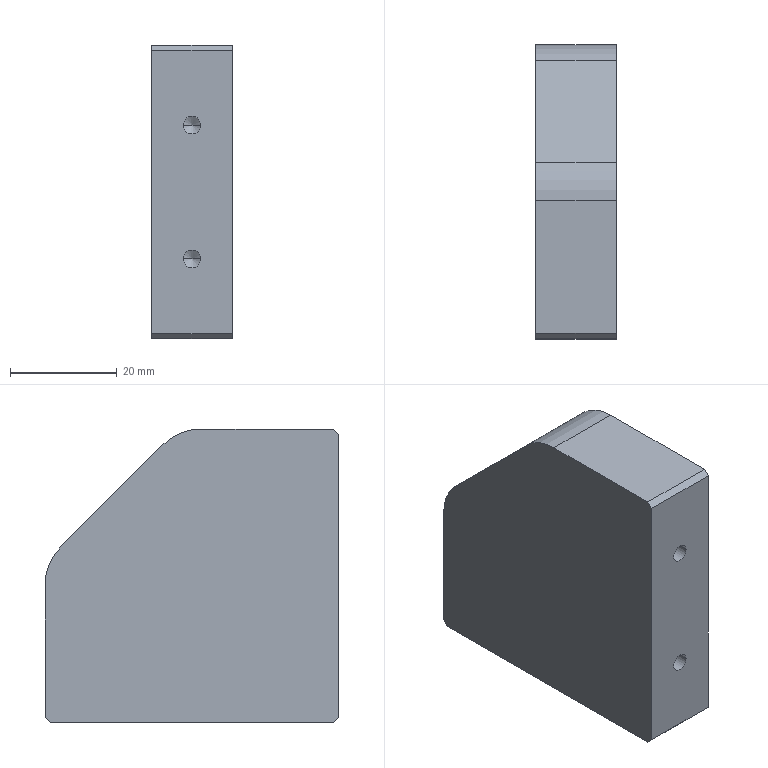Component | SolidWorks | 170423A4-PulleyPlateSupportBlock2-1 | 1 solid | 28 faces | box 15 x 55 x 55 mm | volume 40196 mm3 | cylinder 10 | plane 10 | cone 8 | commonest cylinder face diameters 3.3 x8 20 x2
build123d program:
from build123d import *

# Parameters (mm, degrees)
SKETCH1_W             = 55
SKETCH1_H             = 55
BOSS_EXTRUDE1_DEPTH   = 15
CHAMFER1_SIZE         = 25
M4_TAPPED_HOLE1_D     = 3.3
M4_TAPPED_HOLE1_DEPTH = 11.5
M4_TAPPED_HOLE1_TIP   = 0.9914
M4_TAPPED_HOLE2_D     = 3.3
M4_TAPPED_HOLE2_DEPTH = 11.5
M4_TAPPED_HOLE2_TIP   = 0.9914
FILLET1_R             = 10
CHAMFER2_SIZE         = 1


with BuildPart() as part:
    # Sketch1 → Boss-Extrude1 (new body)
    with BuildSketch(Plane.XY):
        with Locations((27.5, 27.5)):
            Rectangle(SKETCH1_W, SKETCH1_H)
    extrude(amount=BOSS_EXTRUDE1_DEPTH)

    # Chamfer1
    chamfer1_edges = [part.edges().sort_by_distance(p)[0] for p in [
        (55, 55, 7.5),
    ]]
    chamfer(chamfer1_edges, length=CHAMFER1_SIZE)

    # M4 Tapped Hole1
    with Locations(Plane.ZY):
        with Locations((7.5, 40), (7.5, 15)):
            Hole(M4_TAPPED_HOLE1_D / 2, depth=M4_TAPPED_HOLE1_DEPTH)
            with Locations((0, 0, -(M4_TAPPED_HOLE1_DEPTH + M4_TAPPED_HOLE1_TIP / 2))):  # 118° drill point
                Cone(0, M4_TAPPED_HOLE1_D / 2, M4_TAPPED_HOLE1_TIP, mode=Mode.SUBTRACT)

    # M4 Tapped Hole2
    with Locations(Plane(origin=(0, 0, 0), x_dir=(-1, 0, 0), z_dir=(0, -1, 0))):
        with Locations((-15, -7.5), (-40, -7.5)):
            Hole(M4_TAPPED_HOLE2_D / 2, depth=M4_TAPPED_HOLE2_DEPTH)
            with Locations((0, 0, -(M4_TAPPED_HOLE2_DEPTH + M4_TAPPED_HOLE2_TIP / 2))):  # 118° drill point
                Cone(0, M4_TAPPED_HOLE2_D / 2, M4_TAPPED_HOLE2_TIP, mode=Mode.SUBTRACT)

    # Fillet1
    fillet1_edges = [part.edges().sort_by_distance(p)[0] for p in [
        (30, 55, 7.5),
        (55, 30, 7.5),
    ]]
    fillet(fillet1_edges, radius=FILLET1_R)

    # Chamfer2
    chamfer2_edges = [part.edges().sort_by_distance(p)[0] for p in [
        (0, 55, 7.5),
        (55, 0, 7.5),
        (0, 0, 7.5),
    ]]
    chamfer(chamfer2_edges, length=CHAMFER2_SIZE)


solid = part.part

# Placed as in the assembly
solid = solid.moved(Location((-75.246, -163.288, 421), (0, -90, 0)))
STEP:
#1=COLOUR_RGB('',0.7922,0.8196,0.9333);
#2=FILL_AREA_STYLE_COLOUR('',#1);
#3=FILL_AREA_STYLE('',(#2));
#4=SURFACE_STYLE_FILL_AREA(#3);
#5=SURFACE_SIDE_STYLE('',(#4));
#6=SURFACE_STYLE_USAGE(.BOTH.,#5);
#7=PRESENTATION_STYLE_ASSIGNMENT((#6));
#8=CARTESIAN_POINT('',(-3.323,-5.976,18.15));
#9=VERTEX_POINT('',#8);
#10=CARTESIAN_POINT('',(-3.193,-5.976,18.15));
#11=VERTEX_POINT('',#10);
#12=CARTESIAN_POINT('',(-3.258,-5.976,18.15));
#13=DIRECTION('',(0.,-1.,0.));
#14=DIRECTION('',(1.,0.,0.));
#15=AXIS2_PLACEMENT_3D('',#12,#13,#14);
#16=CIRCLE('',#15,0.06496);
#17=EDGE_CURVE('',#9,#11,#16,.T.);
#18=ORIENTED_EDGE('',*,*,#17,.F.);
#19=CARTESIAN_POINT('',(-3.323,-6.429,18.15));
#20=VERTEX_POINT('',#19);
#21=CARTESIAN_POINT('',(-3.323,-6.429,18.15));
#22=DIRECTION('',(0.,-1.,0.));
#23=VECTOR('',#22,39.37);
#24=LINE('',#21,#23);
#25=EDGE_CURVE('',#9,#20,#24,.T.);
#26=ORIENTED_EDGE('',*,*,#25,.T.);
#27=CARTESIAN_POINT('',(-3.193,-6.429,18.15));
#28=VERTEX_POINT('',#27);
#29=CARTESIAN_POINT('',(-3.258,-6.429,18.15));
#30=DIRECTION('',(0.,-1.,0.));
#31=DIRECTION('',(1.,0.,0.));
#32=AXIS2_PLACEMENT_3D('',#29,#30,#31);
#33=CIRCLE('',#32,0.06496);
#34=EDGE_CURVE('',#20,#28,#33,.T.);
#35=ORIENTED_EDGE('',*,*,#34,.T.);
#36=CARTESIAN_POINT('',(-3.193,-6.429,18.15));
#37=DIRECTION('',(0.,-1.,0.));
#38=VECTOR('',#37,39.37);
#39=LINE('',#36,#38);
#40=EDGE_CURVE('',#11,#28,#39,.T.);
#41=ORIENTED_EDGE('',*,*,#40,.F.);
#42=EDGE_LOOP('',(#18,#26,#35,#41));
#43=FACE_OUTER_BOUND('',#42,.T.);
#44=CARTESIAN_POINT('',(-3.258,-6.429,18.15));
#45=DIRECTION('',(0.,-1.,0.));
#46=DIRECTION('',(1.,0.,0.));
#47=AXIS2_PLACEMENT_3D('',#44,#45,#46);
#48=CYLINDRICAL_SURFACE('',#47,0.06496);
#49=ADVANCED_FACE('',(#43),#48,.F.);
#50=CARTESIAN_POINT('',(-3.258,-5.937,18.15));
#51=VERTEX_POINT('',#50);
#52=CARTESIAN_POINT('',(-3.193,-5.976,18.15));
#53=DIRECTION('',(0.8572,-0.515,0.));
#54=VECTOR('',#53,39.37);
#55=LINE('',#52,#54);
#56=EDGE_CURVE('',#51,#11,#55,.T.);
#57=ORIENTED_EDGE('',*,*,#56,.F.);
#58=CARTESIAN_POINT('',(-3.323,-5.976,18.15));
#59=DIRECTION('',(-0.8572,-0.515,0.));
#60=VECTOR('',#59,39.37);
#61=LINE('',#58,#60);
#62=EDGE_CURVE('',#51,#9,#61,.T.);
#63=ORIENTED_EDGE('',*,*,#62,.T.);
#64=ORIENTED_EDGE('',*,*,#17,.T.);
#65=EDGE_LOOP('',(#57,#63,#64));
#66=FACE_OUTER_BOUND('',#65,.T.);
#67=CARTESIAN_POINT('',(-3.258,-5.976,18.15));
#68=DIRECTION('',(0.,-1.,0.));
#69=DIRECTION('',(1.,0.,0.));
#70=AXIS2_PLACEMENT_3D('',#67,#68,#69);
#71=CONICAL_SURFACE('',#70,0.06496,1.03);
#72=ADVANCED_FACE('',(#66),#71,.F.);
#73=CARTESIAN_POINT('',(-3.323,-5.976,17.165));
#74=VERTEX_POINT('',#73);
#75=CARTESIAN_POINT('',(-3.193,-5.976,17.165));
#76=VERTEX_POINT('',#75);
#77=CARTESIAN_POINT('',(-3.258,-5.976,17.165));
#78=DIRECTION('',(0.,-1.,0.));
#79=DIRECTION('',(1.,0.,0.));
#80=AXIS2_PLACEMENT_3D('',#77,#78,#79);
#81=CIRCLE('',#80,0.06496);
#82=EDGE_CURVE('',#74,#76,#81,.T.);
#83=ORIENTED_EDGE('',*,*,#82,.F.);
#84=CARTESIAN_POINT('',(-3.323,-6.429,17.165));
#85=VERTEX_POINT('',#84);
#86=CARTESIAN_POINT('',(-3.323,-6.429,17.165));
#87=DIRECTION('',(0.,-1.,0.));
#88=VECTOR('',#87,39.37);
#89=LINE('',#86,#88);
#90=EDGE_CURVE('',#74,#85,#89,.T.);
#91=ORIENTED_EDGE('',*,*,#90,.T.);
#92=CARTESIAN_POINT('',(-3.193,-6.429,17.165));
#93=VERTEX_POINT('',#92);
#94=CARTESIAN_POINT('',(-3.258,-6.429,17.165));
#95=DIRECTION('',(0.,-1.,0.));
#96=DIRECTION('',(1.,0.,0.));
#97=AXIS2_PLACEMENT_3D('',#94,#95,#96);
#98=CIRCLE('',#97,0.06496);
#99=EDGE_CURVE('',#85,#93,#98,.T.);
#100=ORIENTED_EDGE('',*,*,#99,.T.);
#101=CARTESIAN_POINT('',(-3.193,-6.429,17.165));
#102=DIRECTION('',(0.,-1.,0.));
#103=VECTOR('',#102,39.37);
#104=LINE('',#101,#103);
#105=EDGE_CURVE('',#76,#93,#104,.T.);
#106=ORIENTED_EDGE('',*,*,#105,.F.);
#107=EDGE_LOOP('',(#83,#91,#100,#106));
#108=FACE_OUTER_BOUND('',#107,.T.);
#109=CARTESIAN_POINT('',(-3.258,-6.429,17.165));
#110=DIRECTION('',(0.,-1.,0.));
#111=DIRECTION('',(1.,0.,0.));
#112=AXIS2_PLACEMENT_3D('',#109,#110,#111);
#113=CYLINDRICAL_SURFACE('',#112,0.06496);
#114=ADVANCED_FACE('',(#108),#113,.F.);
#115=CARTESIAN_POINT('',(-3.258,-5.937,17.165));
#116=VERTEX_POINT('',#115);
#117=CARTESIAN_POINT('',(-3.193,-5.976,17.165));
#118=DIRECTION('',(0.8572,-0.515,0.));
#119=VECTOR('',#118,39.37);
#120=LINE('',#117,#119);
#121=EDGE_CURVE('',#116,#76,#120,.T.);
#122=ORIENTED_EDGE('',*,*,#121,.F.);
#123=CARTESIAN_POINT('',(-3.323,-5.976,17.165));
#124=DIRECTION('',(-0.8572,-0.515,0.));
#125=VECTOR('',#124,39.37);
#126=LINE('',#123,#125);
#127=EDGE_CURVE('',#116,#74,#126,.T.);
#128=ORIENTED_EDGE('',*,*,#127,.T.);
#129=ORIENTED_EDGE('',*,*,#82,.T.);
#130=EDGE_LOOP('',(#122,#128,#129));
#131=FACE_OUTER_BOUND('',#130,.T.);
#132=CARTESIAN_POINT('',(-3.258,-5.976,17.165));
#133=DIRECTION('',(0.,-1.,0.));
#134=DIRECTION('',(1.,0.,0.));
#135=AXIS2_PLACEMENT_3D('',#132,#133,#134);
#136=CONICAL_SURFACE('',#135,0.06496,1.03);
#137=ADVANCED_FACE('',(#131),#136,.F.);
#138=CARTESIAN_POINT('',(-3.193,-5.838,17.028));
#139=VERTEX_POINT('',#138);
#140=CARTESIAN_POINT('',(-3.323,-5.838,17.028));
#141=VERTEX_POINT('',#140);
#142=CARTESIAN_POINT('',(-3.258,-5.838,17.028));
#143=DIRECTION('',(0.,0.,-1.));
#144=DIRECTION('',(-1.,0.,0.));
#145=AXIS2_PLACEMENT_3D('',#142,#143,#144);
#146=CIRCLE('',#145,0.06496);
#147=EDGE_CURVE('',#139,#141,#146,.T.);
#148=ORIENTED_EDGE('',*,*,#147,.F.);
#149=CARTESIAN_POINT('',(-3.193,-5.838,16.575));
#150=VERTEX_POINT('',#149);
#151=CARTESIAN_POINT('',(-3.193,-5.838,16.575));
#152=DIRECTION('',(0.,0.,-1.));
#153=VECTOR('',#152,39.37);
#154=LINE('',#151,#153);
#155=EDGE_CURVE('',#139,#150,#154,.T.);
#156=ORIENTED_EDGE('',*,*,#155,.T.);
#157=CARTESIAN_POINT('',(-3.323,-5.838,16.575));
#158=VERTEX_POINT('',#157);
#159=CARTESIAN_POINT('',(-3.258,-5.838,16.575));
#160=DIRECTION('',(0.,0.,-1.));
#161=DIRECTION('',(-1.,0.,0.));
#162=AXIS2_PLACEMENT_3D('',#159,#160,#161);
#163=CIRCLE('',#162,0.06496);
#164=EDGE_CURVE('',#150,#158,#163,.T.);
#165=ORIENTED_EDGE('',*,*,#164,.T.);
#166=CARTESIAN_POINT('',(-3.323,-5.838,16.575));
#167=DIRECTION('',(0.,0.,-1.));
#168=VECTOR('',#167,39.37);
#169=LINE('',#166,#168);
#170=EDGE_CURVE('',#141,#158,#169,.T.);
#171=ORIENTED_EDGE('',*,*,#170,.F.);
#172=EDGE_LOOP('',(#148,#156,#165,#171));
#173=FACE_OUTER_BOUND('',#172,.T.);
#174=CARTESIAN_POINT('',(-3.258,-5.838,16.575));
#175=DIRECTION('',(0.,0.,-1.));
#176=DIRECTION('',(-1.,0.,0.));
#177=AXIS2_PLACEMENT_3D('',#174,#175,#176);
#178=CYLINDRICAL_SURFACE('',#177,0.06496);
#179=ADVANCED_FACE('',(#173),#178,.F.);
#180=CARTESIAN_POINT('',(-3.258,-5.838,17.067));
#181=VERTEX_POINT('',#180);
#182=CARTESIAN_POINT('',(-3.323,-5.838,17.028));
#183=DIRECTION('',(-0.8572,0.,-0.515));
#184=VECTOR('',#183,39.37);
#185=LINE('',#182,#184);
#186=EDGE_CURVE('',#181,#141,#185,.T.);
#187=ORIENTED_EDGE('',*,*,#186,.F.);
#188=CARTESIAN_POINT('',(-3.193,-5.838,17.028));
#189=DIRECTION('',(0.8572,0.,-0.515));
#190=VECTOR('',#189,39.37);
#191=LINE('',#188,#190);
#192=EDGE_CURVE('',#181,#139,#191,.T.);
#193=ORIENTED_EDGE('',*,*,#192,.T.);
#194=ORIENTED_EDGE('',*,*,#147,.T.);
#195=EDGE_LOOP('',(#187,#193,#194));
#196=FACE_OUTER_BOUND('',#195,.T.);
#197=CARTESIAN_POINT('',(-3.258,-5.838,17.028));
#198=DIRECTION('',(0.,0.,-1.));
#199=DIRECTION('',(-1.,0.,0.));
#200=AXIS2_PLACEMENT_3D('',#197,#198,#199);
#201=CONICAL_SURFACE('',#200,0.06496,1.03);
#202=ADVANCED_FACE('',(#196),#201,.F.);
#203=CARTESIAN_POINT('',(-3.193,-4.854,17.028));
#204=VERTEX_POINT('',#203);
#205=CARTESIAN_POINT('',(-3.323,-4.854,17.028));
#206=VERTEX_POINT('',#205);
#207=CARTESIAN_POINT('',(-3.258,-4.854,17.028));
#208=DIRECTION('',(0.,0.,-1.));
#209=DIRECTION('',(-1.,0.,0.));
#210=AXIS2_PLACEMENT_3D('',#207,#208,#209);
#211=CIRCLE('',#210,0.06496);
#212=EDGE_CURVE('',#204,#206,#211,.T.);
#213=ORIENTED_EDGE('',*,*,#212,.F.);
#214=CARTESIAN_POINT('',(-3.193,-4.854,16.575));
#215=VERTEX_POINT('',#214);
#216=CARTESIAN_POINT('',(-3.193,-4.854,16.575));
#217=DIRECTION('',(0.,0.,-1.));
#218=VECTOR('',#217,39.37);
#219=LINE('',#216,#218);
#220=EDGE_CURVE('',#204,#215,#219,.T.);
#221=ORIENTED_EDGE('',*,*,#220,.T.);
#222=CARTESIAN_POINT('',(-3.323,-4.854,16.575));
#223=VERTEX_POINT('',#222);
#224=CARTESIAN_POINT('',(-3.258,-4.854,16.575));
#225=DIRECTION('',(0.,0.,-1.));
#226=DIRECTION('',(-1.,0.,0.));
#227=AXIS2_PLACEMENT_3D('',#224,#225,#226);
#228=CIRCLE('',#227,0.06496);
#229=EDGE_CURVE('',#215,#223,#228,.T.);
#230=ORIENTED_EDGE('',*,*,#229,.T.);
#231=CARTESIAN_POINT('',(-3.323,-4.854,16.575));
#232=DIRECTION('',(0.,0.,-1.));
#233=VECTOR('',#232,39.37);
#234=LINE('',#231,#233);
#235=EDGE_CURVE('',#206,#223,#234,.T.);
#236=ORIENTED_EDGE('',*,*,#235,.F.);
#237=EDGE_LOOP('',(#213,#221,#230,#236));
#238=FACE_OUTER_BOUND('',#237,.T.);
#239=CARTESIAN_POINT('',(-3.258,-4.854,16.575));
#240=DIRECTION('',(0.,0.,-1.));
#241=DIRECTION('',(-1.,0.,0.));
#242=AXIS2_PLACEMENT_3D('',#239,#240,#241);
#243=CYLINDRICAL_SURFACE('',#242,0.06496);
#244=ADVANCED_FACE('',(#238),#243,.F.);
#245=CARTESIAN_POINT('',(-3.258,-4.854,17.067));
#246=VERTEX_POINT('',#245);
#247=CARTESIAN_POINT('',(-3.323,-4.854,17.028));
#248=DIRECTION('',(-0.8572,0.,-0.515));
#249=VECTOR('',#248,39.37);
#250=LINE('',#247,#249);
#251=EDGE_CURVE('',#246,#206,#250,.T.);
#252=ORIENTED_EDGE('',*,*,#251,.F.);
#253=CARTESIAN_POINT('',(-3.193,-4.854,17.028));
#254=DIRECTION('',(0.8572,0.,-0.515));
#255=VECTOR('',#254,39.37);
#256=LINE('',#253,#255);
#257=EDGE_CURVE('',#246,#204,#256,.T.);
#258=ORIENTED_EDGE('',*,*,#257,.T.);
#259=ORIENTED_EDGE('',*,*,#212,.T.);
#260=EDGE_LOOP('',(#252,#258,#259));
#261=FACE_OUTER_BOUND('',#260,.T.);
#262=CARTESIAN_POINT('',(-3.258,-4.854,17.028));
#263=DIRECTION('',(0.,0.,-1.));
#264=DIRECTION('',(-1.,0.,0.));
#265=AXIS2_PLACEMENT_3D('',#262,#263,#264);
#266=CONICAL_SURFACE('',#265,0.06496,1.03);
#267=ADVANCED_FACE('',(#261),#266,.F.);
#268=CARTESIAN_POINT('',(-3.258,-5.838,16.575));
#269=DIRECTION('',(0.,0.,-1.));
#270=DIRECTION('',(-1.,0.,0.));
#271=AXIS2_PLACEMENT_3D('',#268,#269,#270);
#272=CIRCLE('',#271,0.06496);
#273=EDGE_CURVE('',#158,#150,#272,.T.);
#274=ORIENTED_EDGE('',*,*,#273,.F.);
#275=ORIENTED_EDGE('',*,*,#164,.F.);
#276=EDGE_LOOP('',(#274,#275));
#277=FACE_BOUND('',#276,.T.);
#278=CARTESIAN_POINT('',(-3.258,-4.854,16.575));
#279=DIRECTION('',(0.,0.,-1.));
#280=DIRECTION('',(-1.,0.,0.));
#281=AXIS2_PLACEMENT_3D('',#278,#279,#280);
#282=CIRCLE('',#281,0.06496);
#283=EDGE_CURVE('',#223,#215,#282,.T.);
#284=ORIENTED_EDGE('',*,*,#283,.F.);
#285=ORIENTED_EDGE('',*,*,#229,.F.);
#286=EDGE_LOOP('',(#284,#285));
#287=FACE_BOUND('',#286,.T.);
#288=CARTESIAN_POINT('',(-2.962,-4.303,16.575));
#289=VERTEX_POINT('',#288);
#290=CARTESIAN_POINT('',(-2.962,-6.389,16.575));
#291=VERTEX_POINT('',#290);
#292=CARTESIAN_POINT('',(-2.962,-6.429,16.575));
#293=DIRECTION('',(0.,-1.,0.));
#294=VECTOR('',#293,39.37);
#295=LINE('',#292,#294);
#296=EDGE_CURVE('',#289,#291,#295,.T.);
#297=ORIENTED_EDGE('',*,*,#296,.T.);
#298=CARTESIAN_POINT('',(-3.553,-6.389,16.575));
#299=VERTEX_POINT('',#298);
#300=CARTESIAN_POINT('',(-3.553,-6.389,16.575));
#301=DIRECTION('',(-1.,0.,0.));
#302=VECTOR('',#301,39.37);
#303=LINE('',#300,#302);
#304=EDGE_CURVE('',#291,#299,#303,.T.);
#305=ORIENTED_EDGE('',*,*,#304,.T.);
#306=CARTESIAN_POINT('',(-3.553,-4.303,16.575));
#307=VERTEX_POINT('',#306);
#308=CARTESIAN_POINT('',(-3.553,-6.429,16.575));
#309=DIRECTION('',(0.,-1.,0.));
#310=VECTOR('',#309,39.37);
#311=LINE('',#308,#310);
#312=EDGE_CURVE('',#307,#299,#311,.T.);
#313=ORIENTED_EDGE('',*,*,#312,.F.);
#314=CARTESIAN_POINT('',(-3.553,-4.303,16.575));
#315=DIRECTION('',(1.,0.,0.));
#316=VECTOR('',#315,39.37);
#317=LINE('',#314,#316);
#318=EDGE_CURVE('',#307,#289,#317,.T.);
#319=ORIENTED_EDGE('',*,*,#318,.T.);
#320=EDGE_LOOP('',(#297,#305,#313,#319));
#321=FACE_OUTER_BOUND('',#320,.T.);
#322=CARTESIAN_POINT('',(-3.553,-6.429,16.575));
#323=DIRECTION('',(0.,0.,1.));
#324=DIRECTION('',(1.,0.,0.));
#325=AXIS2_PLACEMENT_3D('',#322,#323,#324);
#326=PLANE('',#325);
#327=ADVANCED_FACE('',(#277,#287,#321),#326,.F.);
#328=CARTESIAN_POINT('',(-3.258,-6.429,18.15));
#329=DIRECTION('',(0.,-1.,0.));
#330=DIRECTION('',(1.,0.,0.));
#331=AXIS2_PLACEMENT_3D('',#328,#329,#330);
#332=CIRCLE('',#331,0.06496);
#333=EDGE_CURVE('',#28,#20,#332,.T.);
#334=ORIENTED_EDGE('',*,*,#333,.F.);
#335=ORIENTED_EDGE('',*,*,#34,.F.);
#336=EDGE_LOOP('',(#334,#335));
#337=FACE_BOUND('',#336,.T.);
#338=CARTESIAN_POINT('',(-3.258,-6.429,17.165));
#339=DIRECTION('',(0.,-1.,0.));
#340=DIRECTION('',(1.,0.,0.));
#341=AXIS2_PLACEMENT_3D('',#338,#339,#340);
#342=CIRCLE('',#341,0.06496);
#343=EDGE_CURVE('',#93,#85,#342,.T.);
#344=ORIENTED_EDGE('',*,*,#343,.F.);
#345=ORIENTED_EDGE('',*,*,#99,.F.);
#346=EDGE_LOOP('',(#344,#345));
#347=FACE_BOUND('',#346,.T.);
#348=CARTESIAN_POINT('',(-2.962,-6.429,16.614));
#349=VERTEX_POINT('',#348);
#350=CARTESIAN_POINT('',(-2.962,-6.429,18.701));
#351=VERTEX_POINT('',#350);
#352=CARTESIAN_POINT('',(-2.962,-6.429,16.575));
#353=DIRECTION('',(0.,0.,1.));
#354=VECTOR('',#353,39.37);
#355=LINE('',#352,#354);
#356=EDGE_CURVE('',#349,#351,#355,.T.);
#357=ORIENTED_EDGE('',*,*,#356,.T.);
#358=CARTESIAN_POINT('',(-3.553,-6.429,18.701));
#359=VERTEX_POINT('',#358);
#360=CARTESIAN_POINT('',(-3.553,-6.429,18.701));
#361=DIRECTION('',(-1.,0.,0.));
#362=VECTOR('',#361,39.37);
#363=LINE('',#360,#362);
#364=EDGE_CURVE('',#351,#359,#363,.T.);
#365=ORIENTED_EDGE('',*,*,#364,.T.);
#366=CARTESIAN_POINT('',(-3.553,-6.429,16.614));
#367=VERTEX_POINT('',#366);
#368=CARTESIAN_POINT('',(-3.553,-6.429,16.575));
#369=DIRECTION('',(0.,0.,1.));
#370=VECTOR('',#369,39.37);
#371=LINE('',#368,#370);
#372=EDGE_CURVE('',#367,#359,#371,.T.);
#373=ORIENTED_EDGE('',*,*,#372,.F.);
#374=CARTESIAN_POINT('',(-3.553,-6.429,16.614));
#375=DIRECTION('',(1.,0.,0.));
#376=VECTOR('',#375,39.37);
#377=LINE('',#374,#376);
#378=EDGE_CURVE('',#367,#349,#377,.T.);
#379=ORIENTED_EDGE('',*,*,#378,.T.);
#380=EDGE_LOOP('',(#357,#365,#373,#379));
#381=FACE_OUTER_BOUND('',#380,.T.);
#382=CARTESIAN_POINT('',(-3.553,-6.429,16.575));
#383=DIRECTION('',(0.,1.,0.));
#384=DIRECTION('',(-1.,0.,0.));
#385=AXIS2_PLACEMENT_3D('',#382,#383,#384);
#386=PLANE('',#385);
#387=ADVANCED_FACE('',(#337,#347,#381),#386,.F.);
#388=CARTESIAN_POINT('',(-3.553,-6.389,18.74));
#389=VERTEX_POINT('',#388);
#390=CARTESIAN_POINT('',(-3.553,-5.411,18.74));
#391=VERTEX_POINT('',#390);
#392=CARTESIAN_POINT('',(-3.553,-6.429,18.74));
#393=DIRECTION('',(0.,1.,0.));
#394=VECTOR('',#393,39.37);
#395=LINE('',#392,#394);
#396=EDGE_CURVE('',#389,#391,#395,.T.);
#397=ORIENTED_EDGE('',*,*,#396,.F.);
#398=CARTESIAN_POINT('',(-2.962,-6.389,18.74));
#399=VERTEX_POINT('',#398);
#400=CARTESIAN_POINT('',(-3.553,-6.389,18.74));
#401=DIRECTION('',(1.,0.,0.));
#402=VECTOR('',#401,39.37);
#403=LINE('',#400,#402);
#404=EDGE_CURVE('',#389,#399,#403,.T.);
#405=ORIENTED_EDGE('',*,*,#404,.T.);
#406=CARTESIAN_POINT('',(-2.962,-5.411,18.74));
#407=VERTEX_POINT('',#406);
#408=CARTESIAN_POINT('',(-2.962,-6.429,18.74));
#409=DIRECTION('',(0.,1.,0.));
#410=VECTOR('',#409,39.37);
#411=LINE('',#408,#410);
#412=EDGE_CURVE('',#399,#407,#411,.T.);
#413=ORIENTED_EDGE('',*,*,#412,.T.);
#414=CARTESIAN_POINT('',(-3.553,-5.411,18.74));
#415=DIRECTION('',(-1.,0.,0.));
#416=VECTOR('',#415,39.37);
#417=LINE('',#414,#416);
#418=EDGE_CURVE('',#407,#391,#417,.T.);
#419=ORIENTED_EDGE('',*,*,#418,.T.);
#420=EDGE_LOOP('',(#397,#405,#413,#419));
#421=FACE_OUTER_BOUND('',#420,.T.);
#422=CARTESIAN_POINT('',(-3.553,-6.429,18.74));
#423=DIRECTION('',(0.,0.,-1.));
#424=DIRECTION('',(-1.,0.,0.));
#425=AXIS2_PLACEMENT_3D('',#422,#423,#424);
#426=PLANE('',#425);
#427=ADVANCED_FACE('',(#421),#426,.F.);
#428=CARTESIAN_POINT('',(-2.962,-4.263,17.593));
#429=VERTEX_POINT('',#428);
#430=CARTESIAN_POINT('',(-2.962,-4.263,16.614));
#431=VERTEX_POINT('',#430);
#432=CARTESIAN_POINT('',(-2.962,-4.263,16.575));
#433=DIRECTION('',(0.,0.,-1.));
#434=VECTOR('',#433,39.37);
#435=LINE('',#432,#434);
#436=EDGE_CURVE('',#429,#431,#435,.T.);
#437=ORIENTED_EDGE('',*,*,#436,.T.);
#438=CARTESIAN_POINT('',(-3.553,-4.263,16.614));
#439=VERTEX_POINT('',#438);
#440=CARTESIAN_POINT('',(-3.553,-4.263,16.614));
#441=DIRECTION('',(-1.,0.,0.));
#442=VECTOR('',#441,39.37);
#443=LINE('',#440,#442);
#444=EDGE_CURVE('',#431,#439,#443,.T.);
#445=ORIENTED_EDGE('',*,*,#444,.T.);
#446=CARTESIAN_POINT('',(-3.553,-4.263,17.593));
#447=VERTEX_POINT('',#446);
#448=CARTESIAN_POINT('',(-3.553,-4.263,16.575));
#449=DIRECTION('',(0.,0.,-1.));
#450=VECTOR('',#449,39.37);
#451=LINE('',#448,#450);
#452=EDGE_CURVE('',#447,#439,#451,.T.);
#453=ORIENTED_EDGE('',*,*,#452,.F.);
#454=CARTESIAN_POINT('',(-2.962,-4.263,17.593));
#455=DIRECTION('',(1.,0.,0.));
#456=VECTOR('',#455,39.37);
#457=LINE('',#454,#456);
#458=EDGE_CURVE('',#447,#429,#457,.T.);
#459=ORIENTED_EDGE('',*,*,#458,.T.);
#460=EDGE_LOOP('',(#437,#445,#453,#459));
#461=FACE_OUTER_BOUND('',#460,.T.);
#462=CARTESIAN_POINT('',(-3.553,-4.263,16.575));
#463=DIRECTION('',(0.,-1.,0.));
#464=DIRECTION('',(1.,0.,0.));
#465=AXIS2_PLACEMENT_3D('',#462,#463,#464);
#466=PLANE('',#465);
#467=ADVANCED_FACE('',(#461),#466,.F.);
#468=ORIENTED_EDGE('',*,*,#372,.T.);
#469=CARTESIAN_POINT('',(-3.553,-6.389,18.74));
#470=DIRECTION('',(0.,0.7071,0.7071));
#471=VECTOR('',#470,39.37);
#472=LINE('',#469,#471);
#473=EDGE_CURVE('',#359,#389,#472,.T.);
#474=ORIENTED_EDGE('',*,*,#473,.T.);
#475=ORIENTED_EDGE('',*,*,#396,.T.);
#476=CARTESIAN_POINT('',(-3.553,-5.132,18.625));
#477=VERTEX_POINT('',#476);
#478=CARTESIAN_POINT('',(-3.553,-5.411,18.346));
#479=DIRECTION('',(-1.,0.,0.));
#480=DIRECTION('',(0.,0.,-1.));
#481=AXIS2_PLACEMENT_3D('',#478,#479,#480);
#482=CIRCLE('',#481,0.3937);
#483=EDGE_CURVE('',#391,#477,#482,.T.);
#484=ORIENTED_EDGE('',*,*,#483,.T.);
#485=CARTESIAN_POINT('',(-3.553,-4.379,17.871));
#486=VERTEX_POINT('',#485);
#487=CARTESIAN_POINT('',(-3.553,-4.263,17.756));
#488=DIRECTION('',(0.,0.7071,-0.7071));
#489=VECTOR('',#488,39.37);
#490=LINE('',#487,#489);
#491=EDGE_CURVE('',#477,#486,#490,.T.);
#492=ORIENTED_EDGE('',*,*,#491,.T.);
#493=CARTESIAN_POINT('',(-3.553,-4.657,17.593));
#494=DIRECTION('',(-1.,0.,0.));
#495=DIRECTION('',(0.,-0.,-1.));
#496=AXIS2_PLACEMENT_3D('',#493,#494,#495);
#497=CIRCLE('',#496,0.3937);
#498=EDGE_CURVE('',#486,#447,#497,.T.);
#499=ORIENTED_EDGE('',*,*,#498,.T.);
#500=ORIENTED_EDGE('',*,*,#452,.T.);
#501=CARTESIAN_POINT('',(-3.553,-4.303,16.575));
#502=DIRECTION('',(0.,-0.7071,-0.7071));
#503=VECTOR('',#502,39.37);
#504=LINE('',#501,#503);
#505=EDGE_CURVE('',#439,#307,#504,.T.);
#506=ORIENTED_EDGE('',*,*,#505,.T.);
#507=ORIENTED_EDGE('',*,*,#312,.T.);
#508=CARTESIAN_POINT('',(-3.553,-6.429,16.614));
#509=DIRECTION('',(0.,-0.7071,0.7071));
#510=VECTOR('',#509,39.37);
#511=LINE('',#508,#510);
#512=EDGE_CURVE('',#299,#367,#511,.T.);
#513=ORIENTED_EDGE('',*,*,#512,.T.);
#514=EDGE_LOOP('',(#468,#474,#475,#484,#492,#499,#500,#506,#507,#513));
#515=FACE_OUTER_BOUND('',#514,.T.);
#516=CARTESIAN_POINT('',(-3.553,-6.429,16.575));
#517=DIRECTION('',(1.,0.,0.));
#518=DIRECTION('',(0.,0.,-1.));
#519=AXIS2_PLACEMENT_3D('',#516,#517,#518);
#520=PLANE('',#519);
#521=ADVANCED_FACE('',(#515),#520,.F.);
#522=ORIENTED_EDGE('',*,*,#412,.F.);
#523=CARTESIAN_POINT('',(-2.962,-7.492,17.638));
#524=DIRECTION('',(0.,-0.7071,-0.7071));
#525=VECTOR('',#524,39.37);
#526=LINE('',#523,#525);
#527=EDGE_CURVE('',#399,#351,#526,.T.);
#528=ORIENTED_EDGE('',*,*,#527,.T.);
#529=ORIENTED_EDGE('',*,*,#356,.F.);
#530=CARTESIAN_POINT('',(-2.962,-6.409,16.594));
#531=DIRECTION('',(0.,0.7071,-0.7071));
#532=VECTOR('',#531,39.37);
#533=LINE('',#530,#532);
#534=EDGE_CURVE('',#349,#291,#533,.T.);
#535=ORIENTED_EDGE('',*,*,#534,.T.);
#536=ORIENTED_EDGE('',*,*,#296,.F.);
#537=CARTESIAN_POINT('',(-2.962,-5.366,15.512));
#538=DIRECTION('',(0.,0.7071,0.7071));
#539=VECTOR('',#538,39.37);
#540=LINE('',#537,#539);
#541=EDGE_CURVE('',#289,#431,#540,.T.);
#542=ORIENTED_EDGE('',*,*,#541,.T.);
#543=ORIENTED_EDGE('',*,*,#436,.F.);
#544=CARTESIAN_POINT('',(-2.962,-4.379,17.871));
#545=VERTEX_POINT('',#544);
#546=CARTESIAN_POINT('',(-2.962,-4.657,17.593));
#547=DIRECTION('',(1.,0.,0.));
#548=DIRECTION('',(0.,0.,-1.));
#549=AXIS2_PLACEMENT_3D('',#546,#547,#548);
#550=CIRCLE('',#549,0.3937);
#551=EDGE_CURVE('',#429,#545,#550,.T.);
#552=ORIENTED_EDGE('',*,*,#551,.T.);
#553=CARTESIAN_POINT('',(-2.962,-5.132,18.625));
#554=VERTEX_POINT('',#553);
#555=CARTESIAN_POINT('',(-2.962,-4.755,18.248));
#556=DIRECTION('',(0.,-0.7071,0.7071));
#557=VECTOR('',#556,39.37);
#558=LINE('',#555,#557);
#559=EDGE_CURVE('',#545,#554,#558,.T.);
#560=ORIENTED_EDGE('',*,*,#559,.T.);
#561=CARTESIAN_POINT('',(-2.962,-5.411,18.346));
#562=DIRECTION('',(1.,0.,0.));
#563=DIRECTION('',(0.,0.,-1.));
#564=AXIS2_PLACEMENT_3D('',#561,#562,#563);
#565=CIRCLE('',#564,0.3937);
#566=EDGE_CURVE('',#554,#407,#565,.T.);
#567=ORIENTED_EDGE('',*,*,#566,.T.);
#568=EDGE_LOOP('',(#522,#528,#529,#535,#536,#542,#543,#552,#560,#567));
#569=FACE_OUTER_BOUND('',#568,.T.);
#570=CARTESIAN_POINT('',(-2.962,-6.429,16.575));
#571=DIRECTION('',(1.,0.,0.));
#572=DIRECTION('',(0.,0.,-1.));
#573=AXIS2_PLACEMENT_3D('',#570,#571,#572);
#574=PLANE('',#573);
#575=ADVANCED_FACE('',(#569),#574,.T.);
#576=ORIENTED_EDGE('',*,*,#491,.F.);
#577=CARTESIAN_POINT('',(-2.962,-5.132,18.625));
#578=DIRECTION('',(1.,0.,0.));
#579=VECTOR('',#578,39.37);
#580=LINE('',#577,#579);
#581=EDGE_CURVE('',#477,#554,#580,.T.);
#582=ORIENTED_EDGE('',*,*,#581,.T.);
#583=ORIENTED_EDGE('',*,*,#559,.F.);
#584=CARTESIAN_POINT('',(-3.553,-4.379,17.871));
#585=DIRECTION('',(-1.,0.,0.));
#586=VECTOR('',#585,39.37);
#587=LINE('',#584,#586);
#588=EDGE_CURVE('',#545,#486,#587,.T.);
#589=ORIENTED_EDGE('',*,*,#588,.T.);
#590=EDGE_LOOP('',(#576,#582,#583,#589));
#591=FACE_OUTER_BOUND('',#590,.T.);
#592=CARTESIAN_POINT('',(-3.553,-4.263,17.756));
#593=DIRECTION('',(0.,-0.7071,-0.7071));
#594=DIRECTION('',(1.,0.,0.));
#595=AXIS2_PLACEMENT_3D('',#592,#593,#594);
#596=PLANE('',#595);
#597=ADVANCED_FACE('',(#591),#596,.F.);
#598=ORIENTED_EDGE('',*,*,#257,.F.);
#599=ORIENTED_EDGE('',*,*,#251,.T.);
#600=CARTESIAN_POINT('',(-3.258,-4.854,17.028));
#601=DIRECTION('',(0.,0.,-1.));
#602=DIRECTION('',(-1.,0.,0.));
#603=AXIS2_PLACEMENT_3D('',#600,#601,#602);
#604=CIRCLE('',#603,0.06496);
#605=EDGE_CURVE('',#206,#204,#604,.T.);
#606=ORIENTED_EDGE('',*,*,#605,.T.);
#607=EDGE_LOOP('',(#598,#599,#606));
#608=FACE_OUTER_BOUND('',#607,.T.);
#609=CARTESIAN_POINT('',(-3.258,-4.854,17.028));
#610=DIRECTION('',(0.,0.,-1.));
#611=DIRECTION('',(-1.,0.,0.));
#612=AXIS2_PLACEMENT_3D('',#609,#610,#611);
#613=CONICAL_SURFACE('',#612,0.06496,1.03);
#614=ADVANCED_FACE('',(#608),#613,.F.);
#615=ORIENTED_EDGE('',*,*,#220,.F.);
#616=ORIENTED_EDGE('',*,*,#605,.F.);
#617=ORIENTED_EDGE('',*,*,#235,.T.);
#618=ORIENTED_EDGE('',*,*,#283,.T.);
#619=EDGE_LOOP('',(#615,#616,#617,#618));
#620=FACE_OUTER_BOUND('',#619,.T.);
#621=CARTESIAN_POINT('',(-3.258,-4.854,16.575));
#622=DIRECTION('',(0.,0.,-1.));
#623=DIRECTION('',(-1.,0.,0.));
#624=AXIS2_PLACEMENT_3D('',#621,#622,#623);
#625=CYLINDRICAL_SURFACE('',#624,0.06496);
#626=ADVANCED_FACE('',(#620),#625,.F.);
#627=ORIENTED_EDGE('',*,*,#192,.F.);
#628=ORIENTED_EDGE('',*,*,#186,.T.);
#629=CARTESIAN_POINT('',(-3.258,-5.838,17.028));
#630=DIRECTION('',(0.,0.,-1.));
#631=DIRECTION('',(-1.,0.,0.));
#632=AXIS2_PLACEMENT_3D('',#629,#630,#631);
#633=CIRCLE('',#632,0.06496);
#634=EDGE_CURVE('',#141,#139,#633,.T.);
#635=ORIENTED_EDGE('',*,*,#634,.T.);
#636=EDGE_LOOP('',(#627,#628,#635));
#637=FACE_OUTER_BOUND('',#636,.T.);
#638=CARTESIAN_POINT('',(-3.258,-5.838,17.028));
#639=DIRECTION('',(0.,0.,-1.));
#640=DIRECTION('',(-1.,0.,0.));
#641=AXIS2_PLACEMENT_3D('',#638,#639,#640);
#642=CONICAL_SURFACE('',#641,0.06496,1.03);
#643=ADVANCED_FACE('',(#637),#642,.F.);
#644=ORIENTED_EDGE('',*,*,#155,.F.);
#645=ORIENTED_EDGE('',*,*,#634,.F.);
#646=ORIENTED_EDGE('',*,*,#170,.T.);
#647=ORIENTED_EDGE('',*,*,#273,.T.);
#648=EDGE_LOOP('',(#644,#645,#646,#647));
#649=FACE_OUTER_BOUND('',#648,.T.);
#650=CARTESIAN_POINT('',(-3.258,-5.838,16.575));
#651=DIRECTION('',(0.,0.,-1.));
#652=DIRECTION('',(-1.,0.,0.));
#653=AXIS2_PLACEMENT_3D('',#650,#651,#652);
#654=CYLINDRICAL_SURFACE('',#653,0.06496);
#655=ADVANCED_FACE('',(#649),#654,.F.);
#656=ORIENTED_EDGE('',*,*,#127,.F.);
#657=ORIENTED_EDGE('',*,*,#121,.T.);
#658=CARTESIAN_POINT('',(-3.258,-5.976,17.165));
#659=DIRECTION('',(0.,-1.,0.));
#660=DIRECTION('',(1.,0.,0.));
#661=AXIS2_PLACEMENT_3D('',#658,#659,#660);
#662=CIRCLE('',#661,0.06496);
#663=EDGE_CURVE('',#76,#74,#662,.T.);
#664=ORIENTED_EDGE('',*,*,#663,.T.);
#665=EDGE_LOOP('',(#656,#657,#664));
#666=FACE_OUTER_BOUND('',#665,.T.);
#667=CARTESIAN_POINT('',(-3.258,-5.976,17.165));
#668=DIRECTION('',(0.,-1.,0.));
#669=DIRECTION('',(1.,0.,0.));
#670=AXIS2_PLACEMENT_3D('',#667,#668,#669);
#671=CONICAL_SURFACE('',#670,0.06496,1.03);
#672=ADVANCED_FACE('',(#666),#671,.F.);
#673=ORIENTED_EDGE('',*,*,#90,.F.);
#674=ORIENTED_EDGE('',*,*,#663,.F.);
#675=ORIENTED_EDGE('',*,*,#105,.T.);
#676=ORIENTED_EDGE('',*,*,#343,.T.);
#677=EDGE_LOOP('',(#673,#674,#675,#676));
#678=FACE_OUTER_BOUND('',#677,.T.);
#679=CARTESIAN_POINT('',(-3.258,-6.429,17.165));
#680=DIRECTION('',(0.,-1.,0.));
#681=DIRECTION('',(1.,0.,0.));
#682=AXIS2_PLACEMENT_3D('',#679,#680,#681);
#683=CYLINDRICAL_SURFACE('',#682,0.06496);
#684=ADVANCED_FACE('',(#678),#683,.F.);
#685=ORIENTED_EDGE('',*,*,#62,.F.);
#686=ORIENTED_EDGE('',*,*,#56,.T.);
#687=CARTESIAN_POINT('',(-3.258,-5.976,18.15));
#688=DIRECTION('',(0.,-1.,0.));
#689=DIRECTION('',(1.,0.,0.));
#690=AXIS2_PLACEMENT_3D('',#687,#688,#689);
#691=CIRCLE('',#690,0.06496);
#692=EDGE_CURVE('',#11,#9,#691,.T.);
#693=ORIENTED_EDGE('',*,*,#692,.T.);
#694=EDGE_LOOP('',(#685,#686,#693));
#695=FACE_OUTER_BOUND('',#694,.T.);
#696=CARTESIAN_POINT('',(-3.258,-5.976,18.15));
#697=DIRECTION('',(0.,-1.,0.));
#698=DIRECTION('',(1.,0.,0.));
#699=AXIS2_PLACEMENT_3D('',#696,#697,#698);
#700=CONICAL_SURFACE('',#699,0.06496,1.03);
#701=ADVANCED_FACE('',(#695),#700,.F.);
#702=ORIENTED_EDGE('',*,*,#25,.F.);
#703=ORIENTED_EDGE('',*,*,#692,.F.);
#704=ORIENTED_EDGE('',*,*,#40,.T.);
#705=ORIENTED_EDGE('',*,*,#333,.T.);
#706=EDGE_LOOP('',(#702,#703,#704,#705));
#707=FACE_OUTER_BOUND('',#706,.T.);
#708=CARTESIAN_POINT('',(-3.258,-6.429,18.15));
#709=DIRECTION('',(0.,-1.,0.));
#710=DIRECTION('',(1.,0.,0.));
#711=AXIS2_PLACEMENT_3D('',#708,#709,#710);
#712=CYLINDRICAL_SURFACE('',#711,0.06496);
#713=ADVANCED_FACE('',(#707),#712,.F.);
#714=ORIENTED_EDGE('',*,*,#566,.F.);
#715=ORIENTED_EDGE('',*,*,#581,.F.);
#716=ORIENTED_EDGE('',*,*,#483,.F.);
#717=ORIENTED_EDGE('',*,*,#418,.F.);
#718=EDGE_LOOP('',(#714,#715,#716,#717));
#719=FACE_OUTER_BOUND('',#718,.T.);
#720=CARTESIAN_POINT('',(-3.553,-5.411,18.346));
#721=DIRECTION('',(-1.,0.,0.));
#722=DIRECTION('',(0.,0.,1.));
#723=AXIS2_PLACEMENT_3D('',#720,#721,#722);
#724=CYLINDRICAL_SURFACE('',#723,0.3937);
#725=ADVANCED_FACE('',(#719),#724,.T.);
#726=ORIENTED_EDGE('',*,*,#498,.F.);
#727=ORIENTED_EDGE('',*,*,#588,.F.);
#728=ORIENTED_EDGE('',*,*,#551,.F.);
#729=ORIENTED_EDGE('',*,*,#458,.F.);
#730=EDGE_LOOP('',(#726,#727,#728,#729));
#731=FACE_OUTER_BOUND('',#730,.T.);
#732=CARTESIAN_POINT('',(-3.553,-4.657,17.593));
#733=DIRECTION('',(1.,0.,0.));
#734=DIRECTION('',(0.,0.,-1.));
#735=AXIS2_PLACEMENT_3D('',#732,#733,#734);
#736=CYLINDRICAL_SURFACE('',#735,0.3937);
#737=ADVANCED_FACE('',(#731),#736,.T.);
#738=ORIENTED_EDGE('',*,*,#473,.F.);
#739=ORIENTED_EDGE('',*,*,#364,.F.);
#740=ORIENTED_EDGE('',*,*,#527,.F.);
#741=ORIENTED_EDGE('',*,*,#404,.F.);
#742=EDGE_LOOP('',(#738,#739,#740,#741));
#743=FACE_OUTER_BOUND('',#742,.T.);
#744=CARTESIAN_POINT('',(-3.553,-6.389,18.74));
#745=DIRECTION('',(0.,0.7071,-0.7071));
#746=DIRECTION('',(1.,0.,0.));
#747=AXIS2_PLACEMENT_3D('',#744,#745,#746);
#748=PLANE('',#747);
#749=ADVANCED_FACE('',(#743),#748,.F.);
#750=ORIENTED_EDGE('',*,*,#512,.F.);
#751=ORIENTED_EDGE('',*,*,#304,.F.);
#752=ORIENTED_EDGE('',*,*,#534,.F.);
#753=ORIENTED_EDGE('',*,*,#378,.F.);
#754=EDGE_LOOP('',(#750,#751,#752,#753));
#755=FACE_OUTER_BOUND('',#754,.T.);
#756=CARTESIAN_POINT('',(-3.553,-6.429,16.614));
#757=DIRECTION('',(0.,0.7071,0.7071));
#758=DIRECTION('',(1.,0.,0.));
#759=AXIS2_PLACEMENT_3D('',#756,#757,#758);
#760=PLANE('',#759);
#761=ADVANCED_FACE('',(#755),#760,.F.);
#762=ORIENTED_EDGE('',*,*,#505,.F.);
#763=ORIENTED_EDGE('',*,*,#444,.F.);
#764=ORIENTED_EDGE('',*,*,#541,.F.);
#765=ORIENTED_EDGE('',*,*,#318,.F.);
#766=EDGE_LOOP('',(#762,#763,#764,#765));
#767=FACE_OUTER_BOUND('',#766,.T.);
#768=CARTESIAN_POINT('',(-3.553,-4.303,16.575));
#769=DIRECTION('',(0.,-0.7071,0.7071));
#770=DIRECTION('',(1.,0.,0.));
#771=AXIS2_PLACEMENT_3D('',#768,#769,#770);
#772=PLANE('',#771);
#773=ADVANCED_FACE('',(#767),#772,.F.);
#774=CLOSED_SHELL('',(#49,#72,#114,#137,#179,#202,#244,#267,#327,#387,#427,#467,#521,#575,#597,#614,#626,#643,#655,#672,#684,#701,#713,#725,#737,#749,#761,#773));
#775=MANIFOLD_SOLID_BREP('',#774);
#776=STYLED_ITEM('',(#7),#775);
#777=(LENGTH_UNIT()NAMED_UNIT(*)SI_UNIT($,.METRE.));
#778=LENGTH_MEASURE_WITH_UNIT(LENGTH_MEASURE(0.0254),#777);
#779=DIMENSIONAL_EXPONENTS(1.,0.,0.,0.,0.,0.,0.);
#780=(CONVERSION_BASED_UNIT('',#778)LENGTH_UNIT()NAMED_UNIT(#779));
#781=UNCERTAINTY_MEASURE_WITH_UNIT(LENGTH_MEASURE(0.00001),#780,'','');
#782=(NAMED_UNIT(*)PLANE_ANGLE_UNIT()SI_UNIT($,.RADIAN.));
#783=(NAMED_UNIT(*)SI_UNIT($,.STERADIAN.)SOLID_ANGLE_UNIT());
#784=(GEOMETRIC_REPRESENTATION_CONTEXT(3)GLOBAL_UNCERTAINTY_ASSIGNED_CONTEXT((#781))GLOBAL_UNIT_ASSIGNED_CONTEXT((#780,#782,#783))REPRESENTATION_CONTEXT('',''));
#785=MECHANICAL_DESIGN_GEOMETRIC_PRESENTATION_REPRESENTATION('',(#776),#784);
#786=CARTESIAN_POINT('',(0.,0.,0.));
#787=DIRECTION('',(0.,0.,1.));
#788=DIRECTION('',(1.,0.,0.));
#789=AXIS2_PLACEMENT_3D('',#786,#787,#788);
#790=(LENGTH_UNIT()NAMED_UNIT(*)SI_UNIT($,.METRE.));
#791=LENGTH_MEASURE_WITH_UNIT(LENGTH_MEASURE(0.0254),#790);
#792=DIMENSIONAL_EXPONENTS(1.,0.,0.,0.,0.,0.,0.);
#793=(CONVERSION_BASED_UNIT('',#791)LENGTH_UNIT()NAMED_UNIT(#792));
#794=UNCERTAINTY_MEASURE_WITH_UNIT(LENGTH_MEASURE(0.00001),#793,'','');
#795=(NAMED_UNIT(*)PLANE_ANGLE_UNIT()SI_UNIT($,.RADIAN.));
#796=(NAMED_UNIT(*)SI_UNIT($,.STERADIAN.)SOLID_ANGLE_UNIT());
#797=(GEOMETRIC_REPRESENTATION_CONTEXT(3)GLOBAL_UNCERTAINTY_ASSIGNED_CONTEXT((#794))GLOBAL_UNIT_ASSIGNED_CONTEXT((#793,#795,#796))REPRESENTATION_CONTEXT('',''));
#798=ADVANCED_BREP_SHAPE_REPRESENTATION('',(#775,#789),#797);
#799=PRESENTATION_LAYER_ASSIGNMENT('','',(#776));